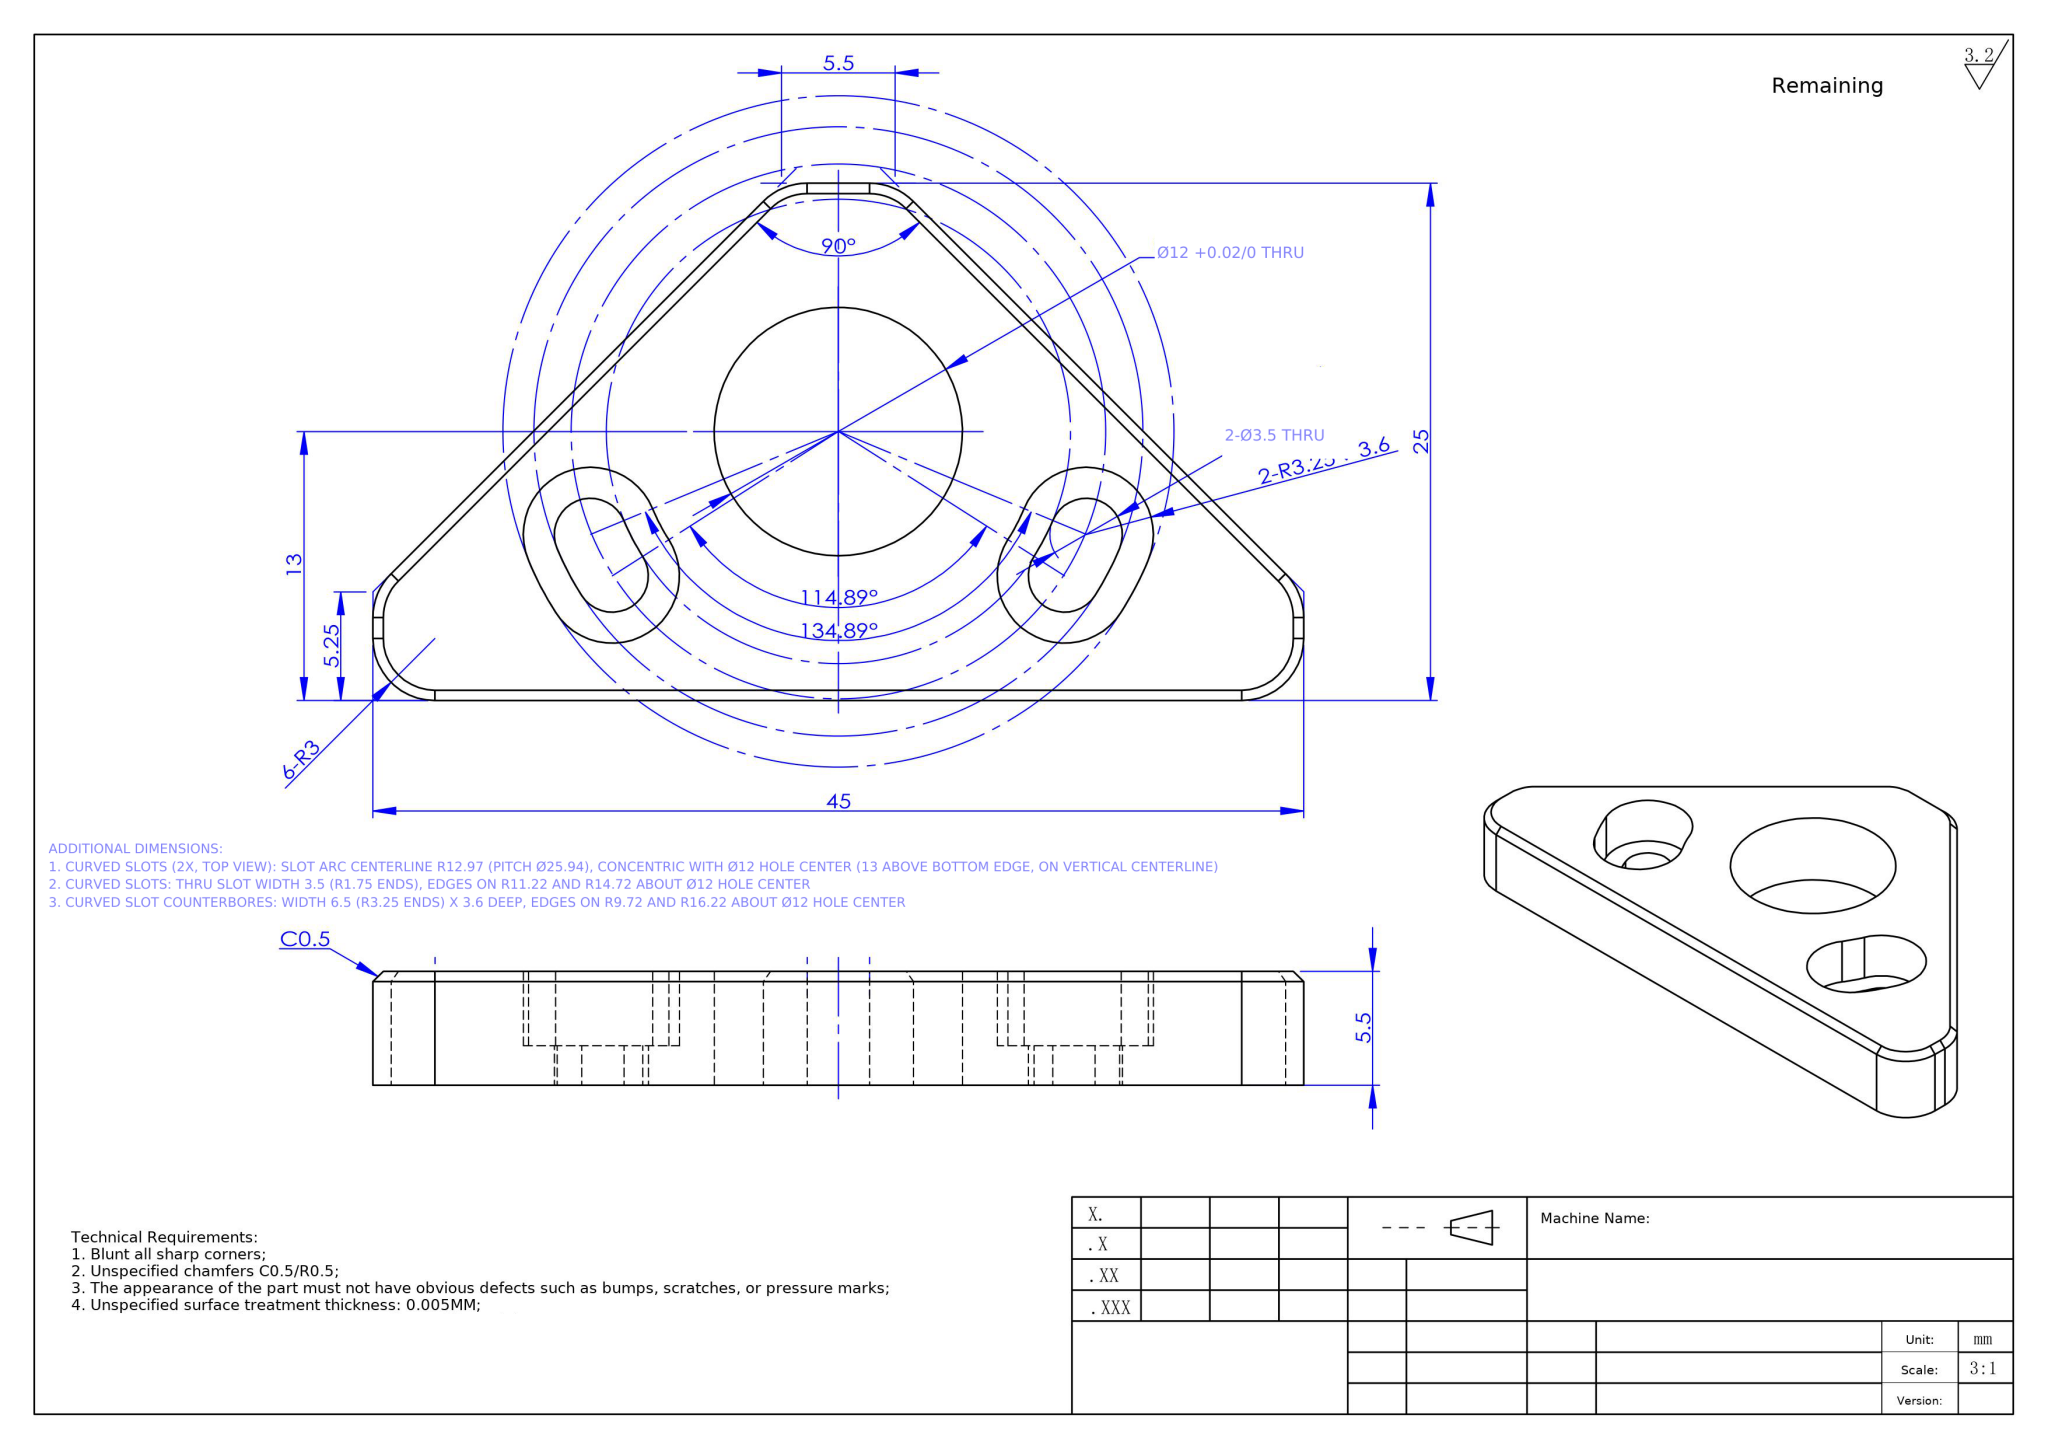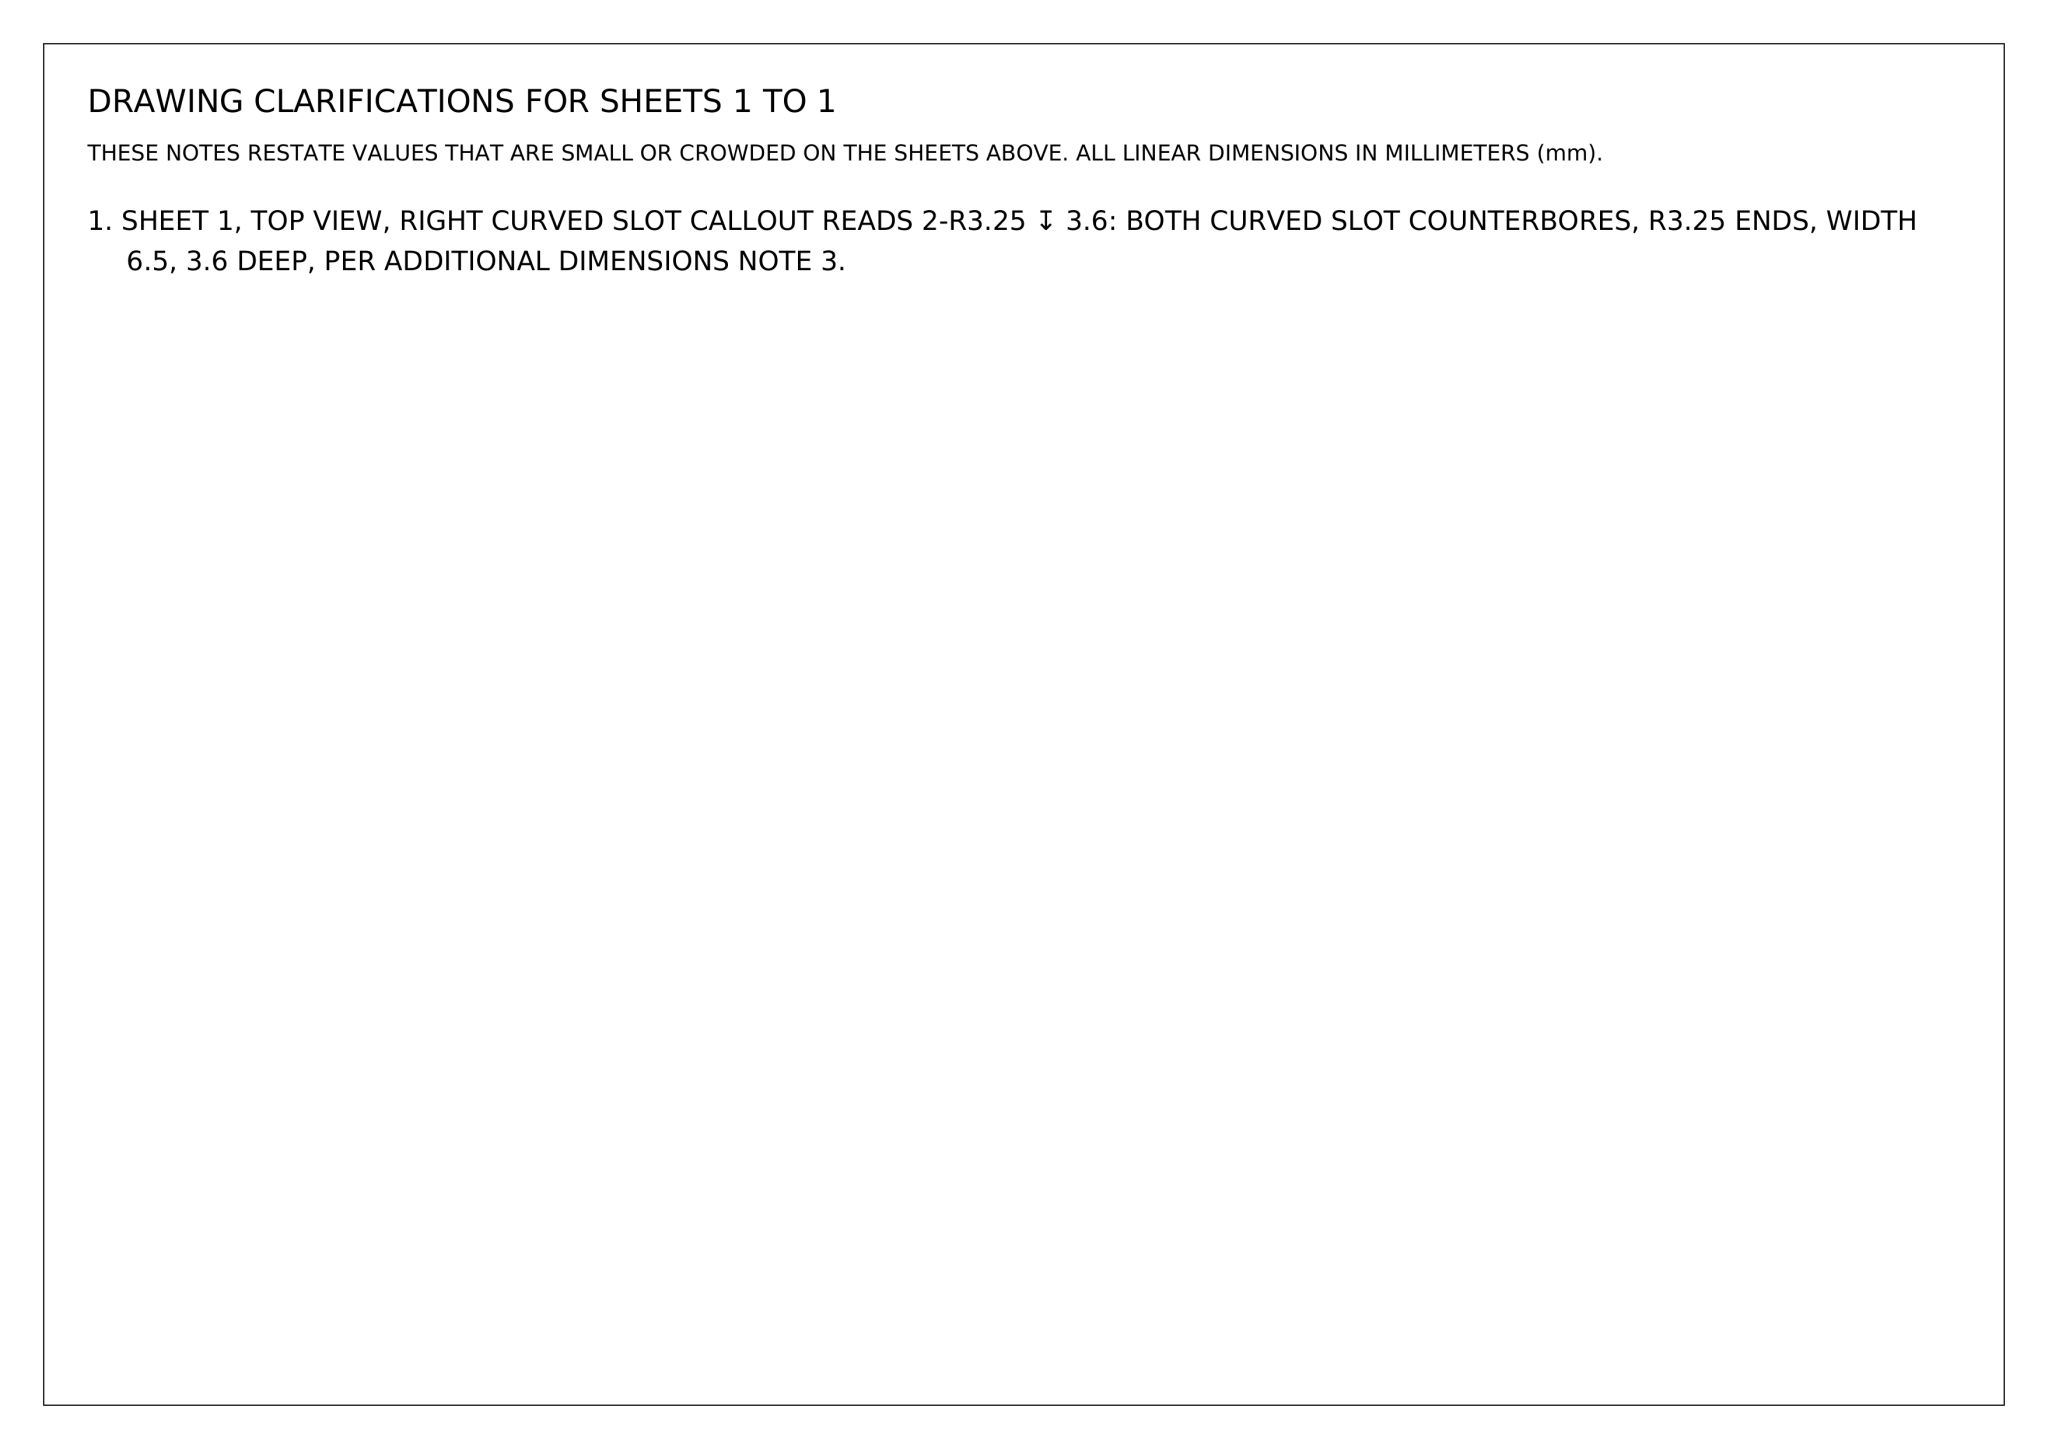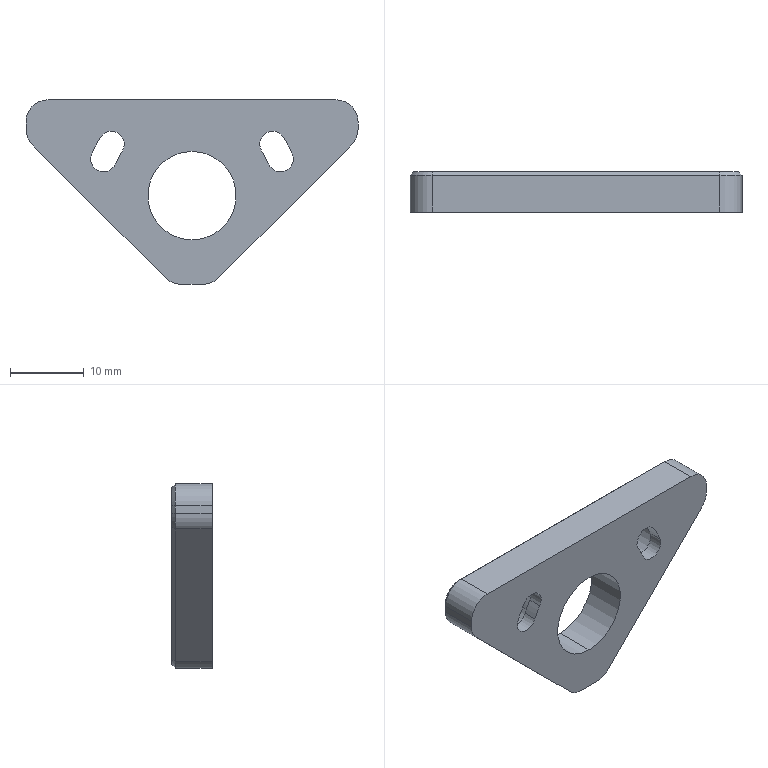Part | NX | mm | 1 solid | 50 faces | box 45 x 5.5 x 25 mm | volume 2969 mm3 | cylinder 28 | plane 16 | cone 6 | commonest cylinder face diameters 6.5 x6 3.5 x6 6 x6 12 x2 22.442 x2 29.442 x2 19.442 x2 32.442 x2